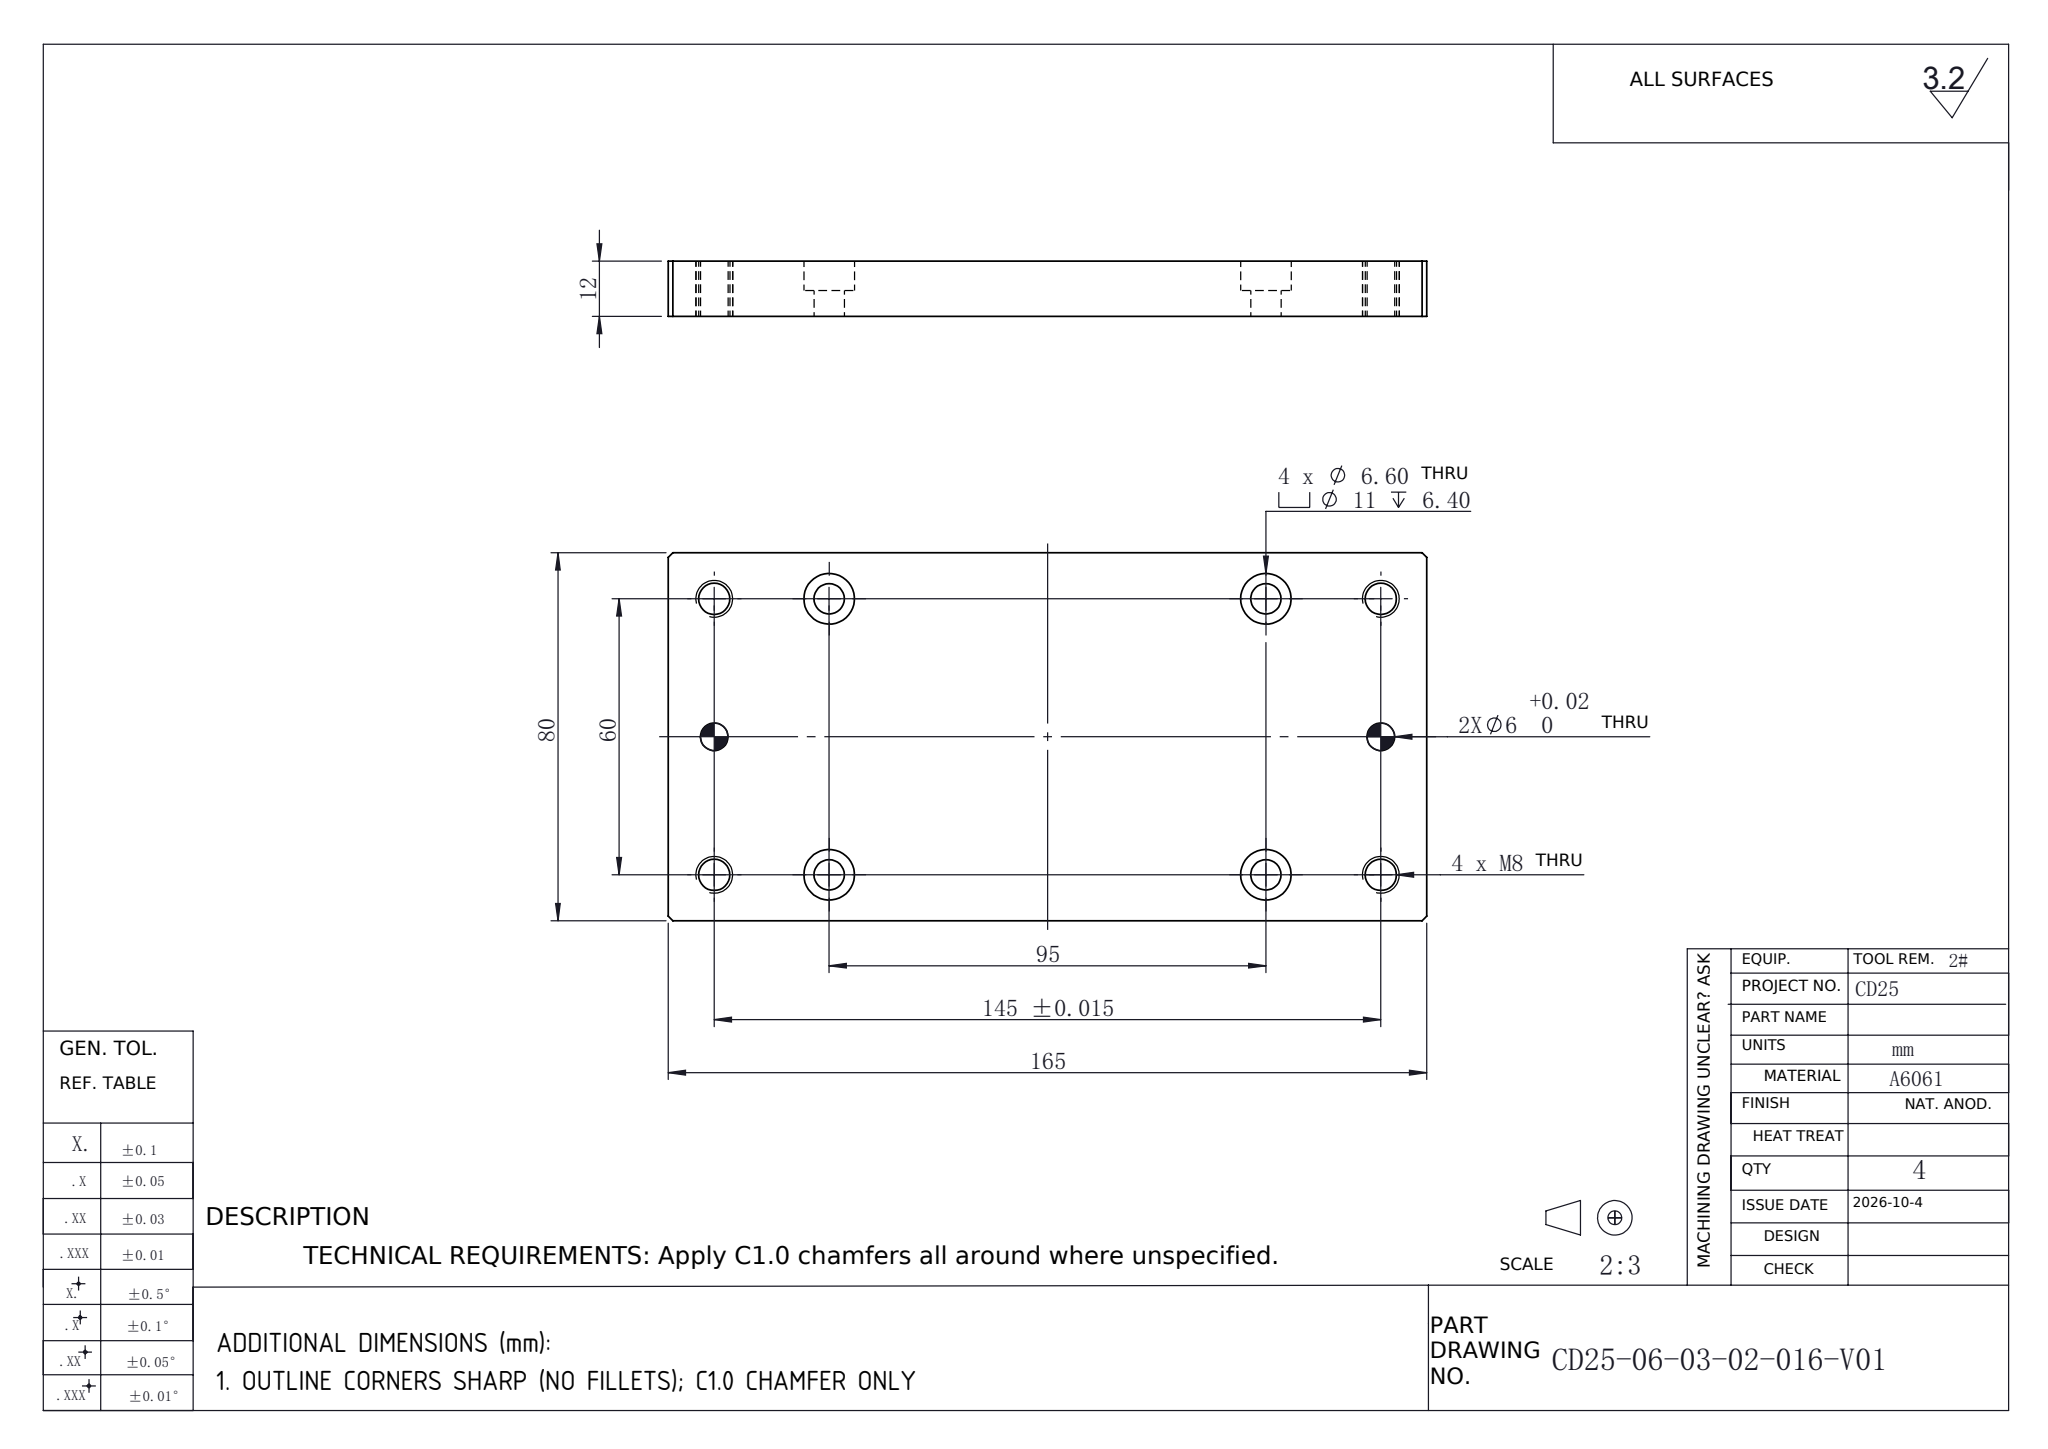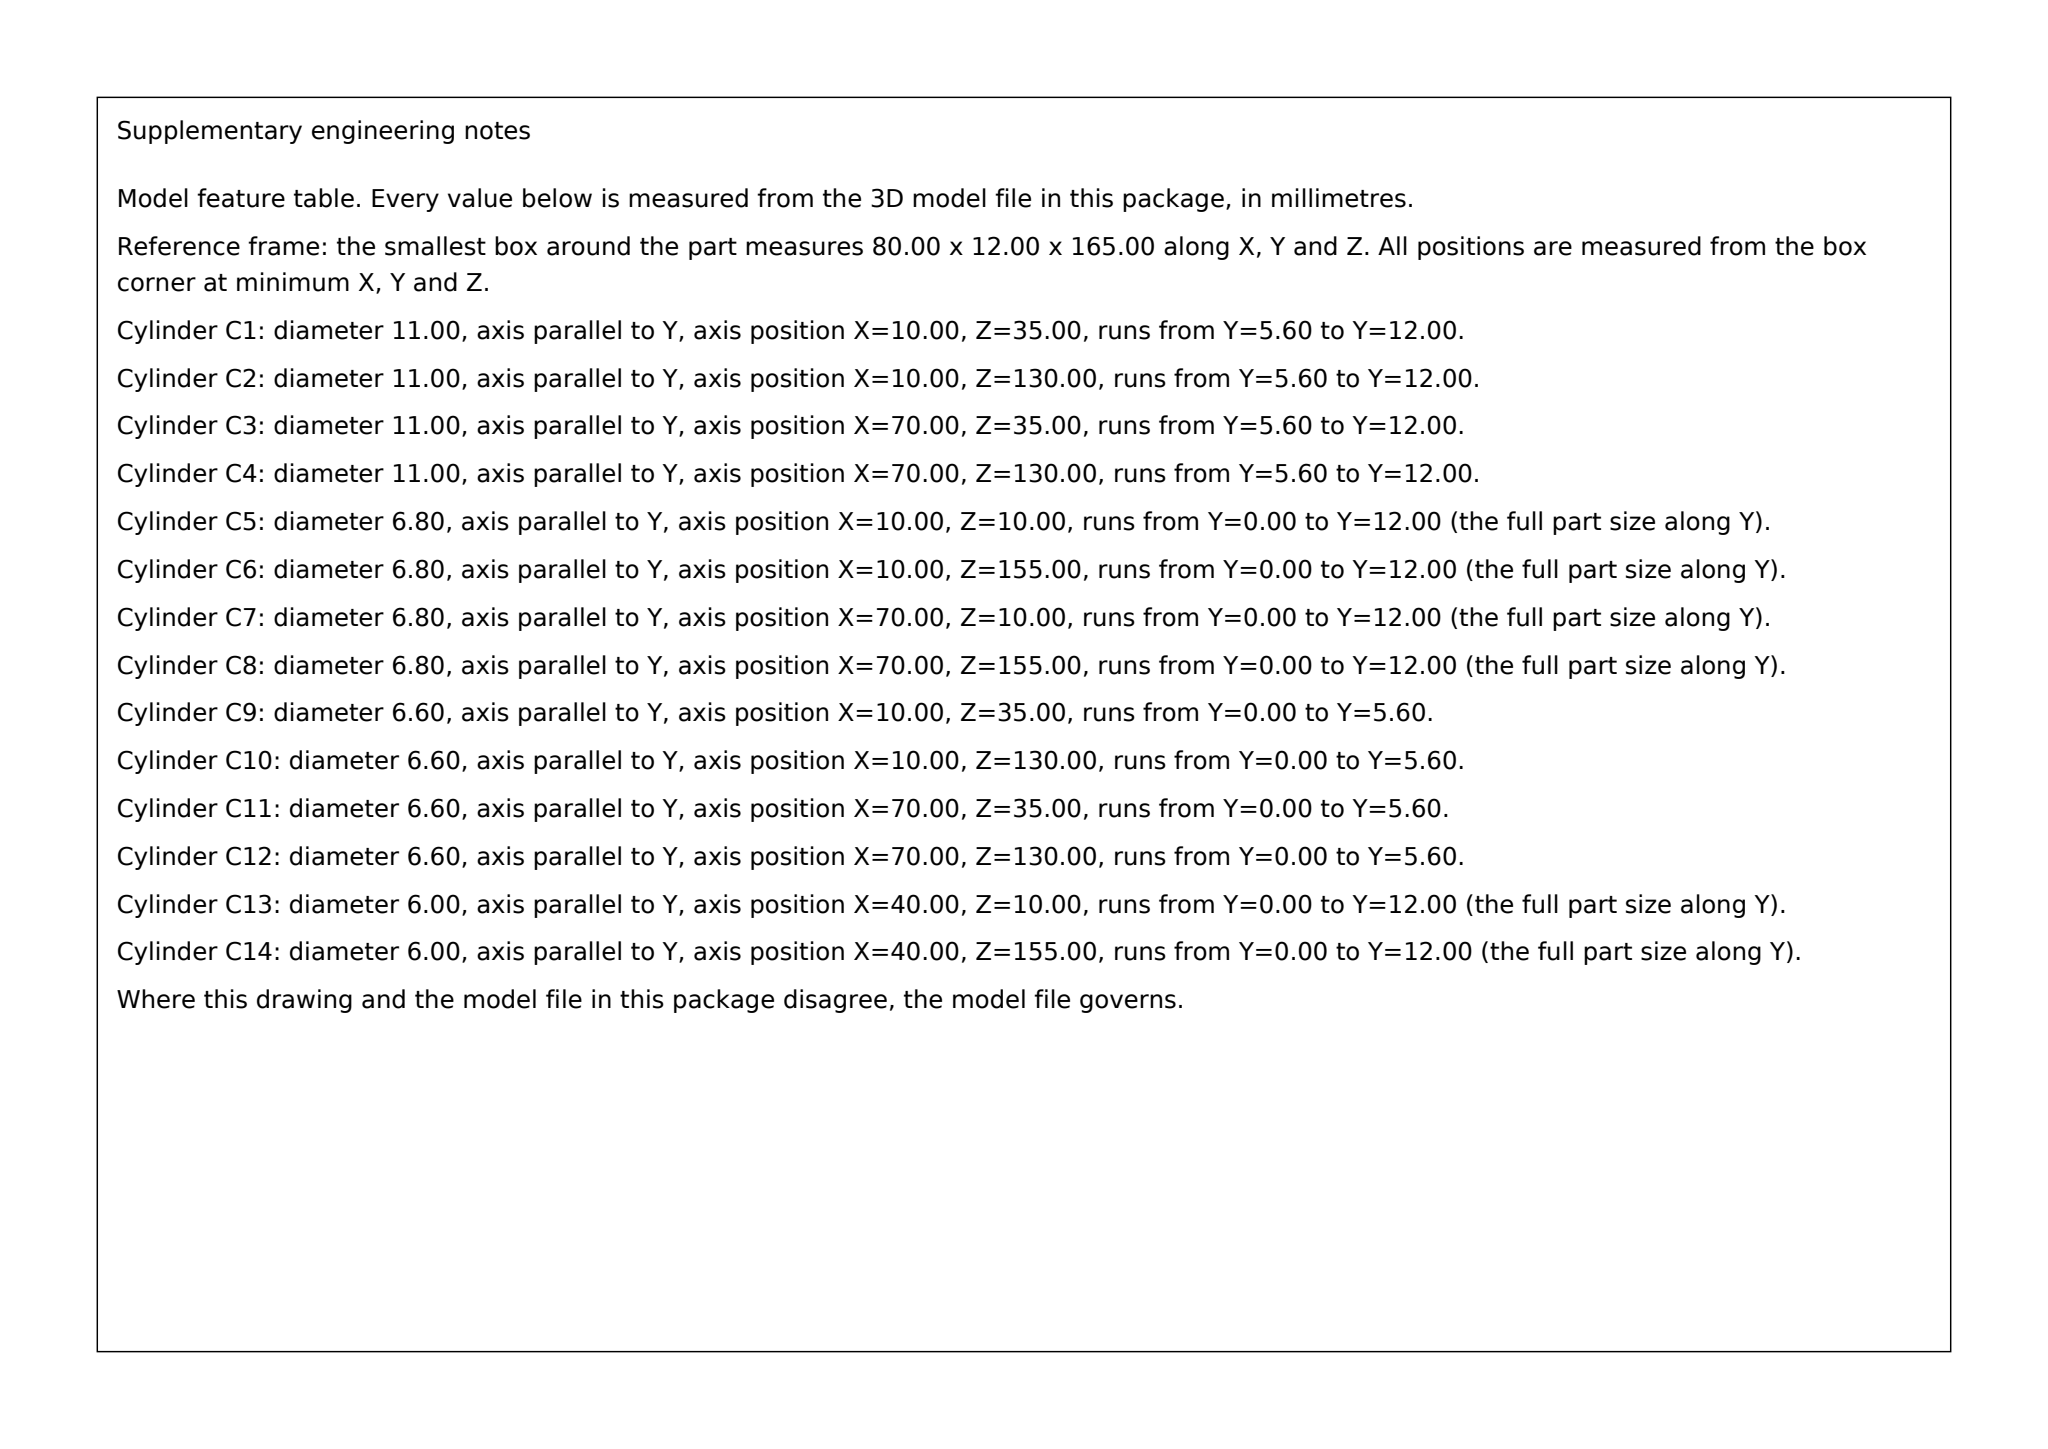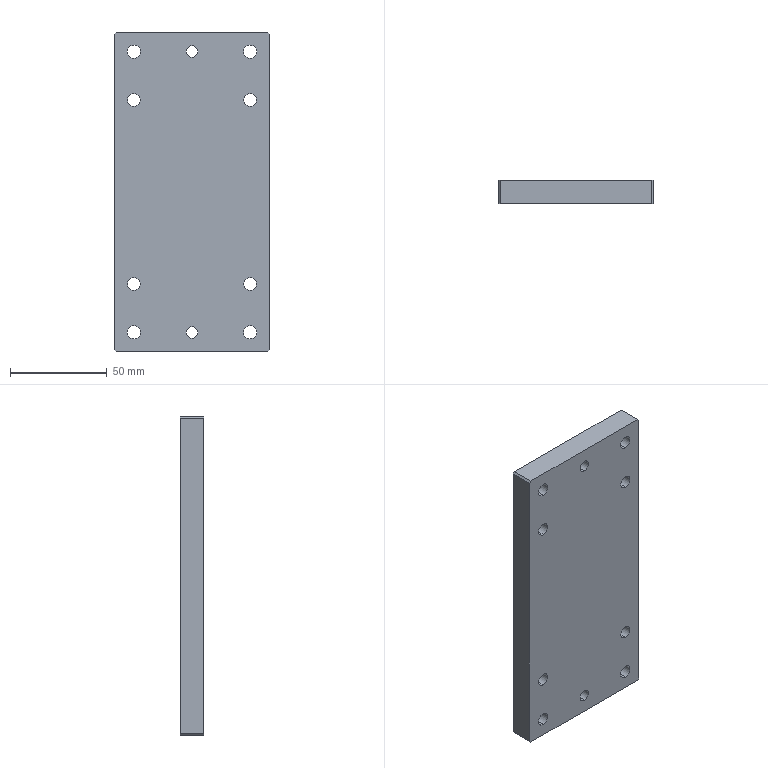Part | SolidWorks | mm | 1 solid | 42 faces | box 80 x 12 x 165 mm | volume 152755 mm3 | cylinder 28 | plane 14 | commonest cylinder face diameters 11 x8 6.6 x8 6.8 x8 6 x4
build123d program:
from build123d import *

# Parameters (mm, degrees)
SKETCH1_W                                       = 80
SKETCH1_H                                       = 165
BOSS_EXTRUDE1_DEPTH                             = 6
M8_TAPPED_HOLE1_D                               = 6.8
CHAMFER1_SIZE                                   = 1
F_6_0MM_DOWEL_PIN_HOLE1_D                       = 6
M6_HEX_SOCKET_HEAD_CAP_SCREW_CBORE1_D           = 6.6
M6_HEX_SOCKET_HEAD_CAP_SCREW_CBORE1_CBORE_D     = 11
M6_HEX_SOCKET_HEAD_CAP_SCREW_CBORE1_CBORE_DEPTH = 6.4


with BuildPart() as part:
    # Sketch1 → Boss-Extrude1 (new, symmetric)
    with BuildSketch(Plane(origin=(0, 0, 0), x_dir=(1, 0, 0), z_dir=(0, 1, 0))):
        Rectangle(SKETCH1_W, SKETCH1_H)
    extrude(amount=BOSS_EXTRUDE1_DEPTH, both=True)

    # M8 Tapped Hole1 (through all)
    with Locations(Plane(origin=(0, 6, 0), x_dir=(1, 0, 0), z_dir=(0, 1, 0))):
        with Locations((-30, 72.5), (30, 72.5), (30, -72.5), (-30, -72.5)):
            Hole(M8_TAPPED_HOLE1_D / 2)

    # Chamfer1
    chamfer1_edges = [part.edges().sort_by_distance(p)[0] for p in [
        (40, 0, 82.5),
        (-40, 0, 82.5),
        (-40, 0, -82.5),
        (40, 0, -82.5),
    ]]
    chamfer(chamfer1_edges, length=CHAMFER1_SIZE)

    # 6.0mm Dowel Pin Hole1 (through all)
    with Locations(Plane(origin=(0, 6, 0), x_dir=(1, 0, 0), z_dir=(0, 1, 0))):
        with Locations((0, -72.5), (0, 72.5)):
            Hole(F_6_0MM_DOWEL_PIN_HOLE1_D / 2)

    # M6 Hex Socket Head Cap Screw CBORE1 (through all)
    with Locations(Plane(origin=(0, 6, 0), x_dir=(1, 0, 0), z_dir=(0, 1, 0))):
        with Locations((-30, 47.5), (-30, -47.5), (30, -47.5), (30, 47.5)):
            CounterBoreHole(M6_HEX_SOCKET_HEAD_CAP_SCREW_CBORE1_D / 2, M6_HEX_SOCKET_HEAD_CAP_SCREW_CBORE1_CBORE_D / 2, M6_HEX_SOCKET_HEAD_CAP_SCREW_CBORE1_CBORE_DEPTH)


solid = part.part